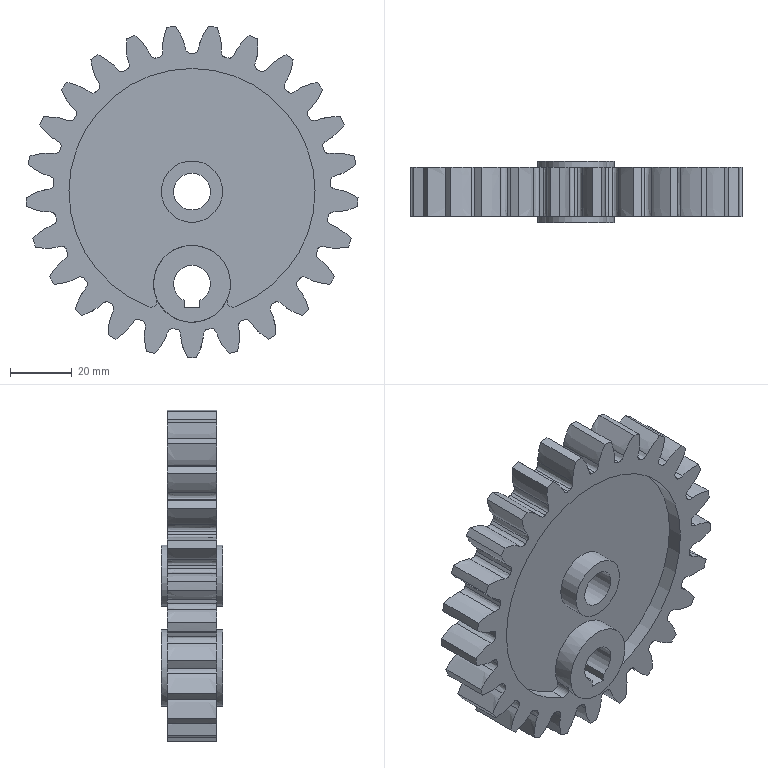Component | NX | ECCENTRIC_GEAR | 1 solid | 173 faces | volume 80127 mm3 | other 125 | cylinder 37 | plane 11 | commonest cylinder face diameters 90 x25 4 x4 80 x2 20 x2 12 x2 25 x2